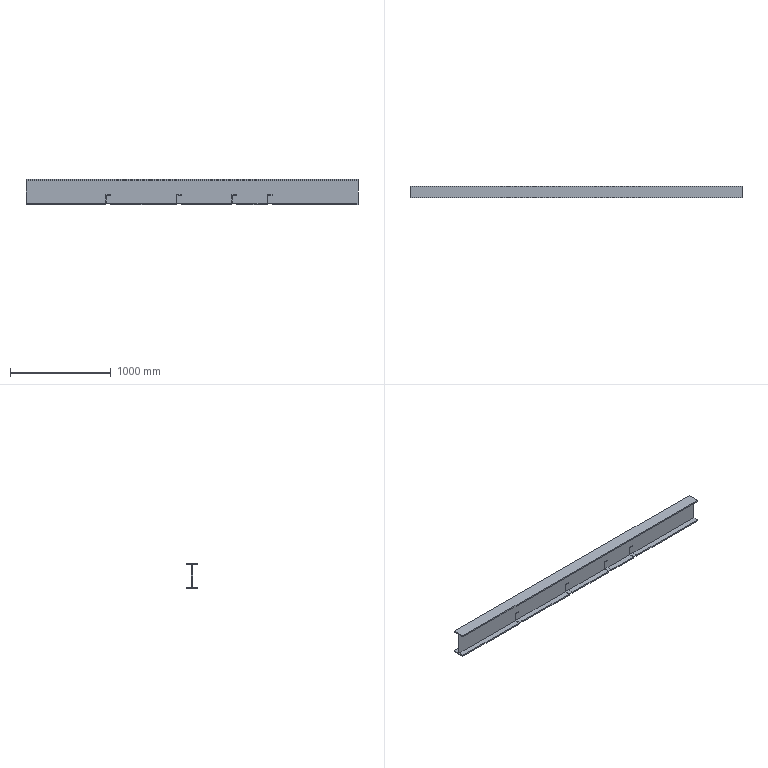Component | NX | CHUNSHUIJINCAO_1 | 1 solid | 62 faces | volume 17231833 mm3 | plane 62